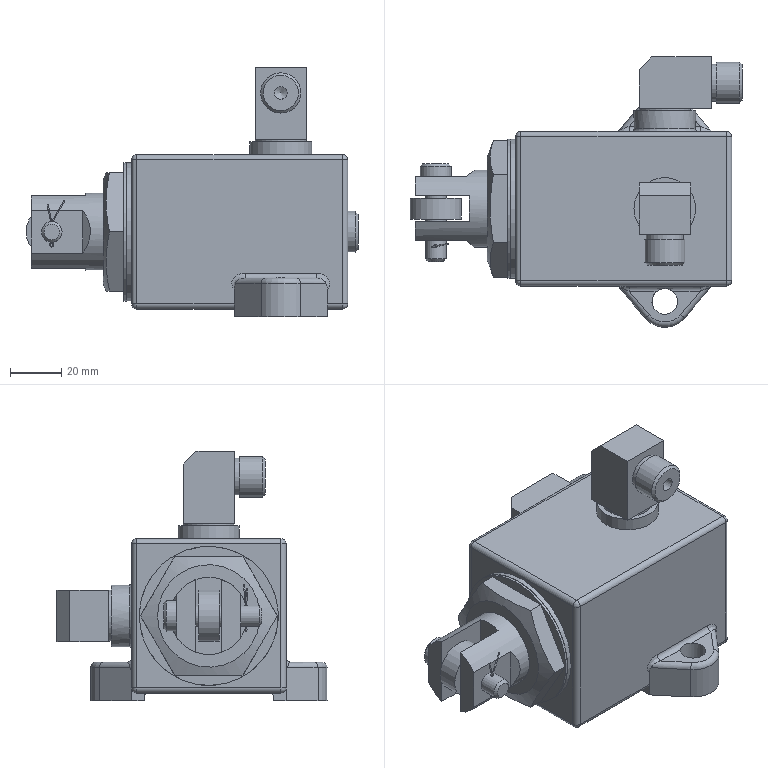Assembly | NX | mm | 18 component files | 18 solids | 273 faces | box 129 x 105 x 97 mm | volume 309682 mm3 | plane 129 | cylinder 84 | spline 26 | cone 21 | sphere 10 | torus 3 | commonest cylinder face diameters 4 x20 5 x6 8 x6 20 x5 3.2 x4 14.5 x4 16 x4 30 x4
Bill of materials:
unnamed part 1 | 2 |  | Short thick-walled cylindrical sleeve with a central through bore and a straight rectangular slot cut across one end face, running through the bore and partway along the length.
unnamed part 2 | 1 |  | Headed cylindrical pin: a plain shank with a larger cylindrical head at one end, chamfers on both ends, and a small cross hole through the shank near the free end.
unnamed part 3 | 2 |  | Rectangular block with one beveled corner. A stepped cylindrical boss sticks out of one side face, and a second stepped cylindrical boss sticks out of the bottom face at a right angle to the first, giving an L-shaped (elbow-like) form.
unnamed part 4 | 1 |  | Cylindrical tubular body with a thin flange at one end and a bore opening at that end. The other end is slotted into a two-tongue fork, and the tongues have a transverse cross hole. The outer surface has two narrow circumferential grooves and a tapered step at the slotted end.
unnamed part 5 | 1 |  | Hollow, stepped bushing-like part. It has a hexagonal collar at one end, a thin round flange next to the hex, a larger cylindrical step, and a smaller cylindrical spigot. A through bore runs the full length.
unnamed part 6 | 1 |  | Helical coil of round wire forming a cylindrical, open-coil spring shape with roughly constant pitch and diameter. One end coil appears flattened or ground.
unnamed part 7 | 1 |  | Thin flat annular ring (washer-like) with a large central opening compared with its outer diameter.
unnamed part 8 | 1 |  | Bent round wire formed into a loop eye at one end, with two parallel legs that run side by side and then splay apart at an angle toward their free ends.
unnamed part 9 | 1 |  | Thick plain cylindrical ring or spacer with a concentric through bore and square, unchamfered edges.
unnamed part 10 | 2 |  | Thin flat annular ring with a large central opening and moderate radial width.
unnamed part 11 | 1 |  | Open-pitch cylindrical helical coil of round wire with roughly uniform diameter and pitch along its length.
unnamed part 12 | 2 |  | Solid headed pin with a domed (hemispherical-type) head and a plain cylindrical shank with a flat end.
unnamed part 13 | 1 |  | Rectangular box-shaped body with rounded edges. It has a short cylindrical boss with a through or blind bore on one face, a second cylindrical boss sticking out of a side face, and two tapered, rounded mounting tabs with holes on opposite sides at the base.
unnamed part 14 | 1 |  | Helical coil spring with constant diameter and roughly eight evenly spaced open coils. The coil end looks flat, giving a flat ring-shaped face in the end view.
Mates:
1. fix | pump_body 1 component
2. touch align | SPRING_CYLINDER_COMPRESSION_1 1 datumaxis | pump_body 1 face
3. touch align | SPRING_CYLINDER_COMPRESSION_1 1 face | pump_body 1 face
4. touch align | plunger 1 face | pump_body 1 face
5. touch align | plunger 1 face | SPRING_CYLINDER_COMPRESSION_1 1 face
6. concentric | large_washer 1 arc | pump_body 1 edge
7. concentric | plunger_sleeve 1 edge | large_washer 1 edge
8. parallel | plunger_sleeve 1 face | pump_body 1 face
9. concentric | shaft 1 edge | plunger 1 edge
10. touch align | idler_wheel 1 face | shaft 1 face
11. center | idler_wheel 1 face | idler_wheel 1 face | plunger 1 face | plunger 1 face
12. center | pin 1 line | pin 1 line | shaft 1 face
13. fix | pin 1 component
14. concentric | small_washer 2 arc | pump_body 1 edge
15. concentric | small_washer 1 arc | pump_body 1 edge
16. concentric | check_valve_body 2 arc | small_washer 2 edge
17. parallel | check_valve_body 2 face | pump_body 1 face
18. concentric | check_valve_body 1 arc | small_washer 1 edge
19. parallel | check_valve_body 1 face | pump_body 1 face
20. touch align | valve_ball 2 face | check_valve_body 1 face
21. touch align | valve_ball 2 face | check_valve_body 1 face
22. touch align | SPRING_CYLINDER_COMPRESSION_2 2 datumaxis | check_valve_body 1 face
23. touch align | valve_ball 2 face | SPRING_CYLINDER_COMPRESSION_2 2 face
24. touch align | holed_plug 2 face | check_valve_body 1 face
25. touch align | SPRING_CYLINDER_COMPRESSION_2 2 face | holed_plug 2 face
26. touch align | valve_ball 1 face | check_valve_body 2 face
27. touch align | valve_ball 1 face | check_valve_body 2 face
28. touch align | SPRING_CYLINDER_COMPRESSION_2 1 datumaxis | valve_ball 1 face
29. touch align | SPRING_CYLINDER_COMPRESSION_2 1 face | valve_ball 1 face
30. touch align | holed_plug 1 face | check_valve_body 2 face
31. touch align | SPRING_CYLINDER_COMPRESSION_2 1 face | holed_plug 1 face